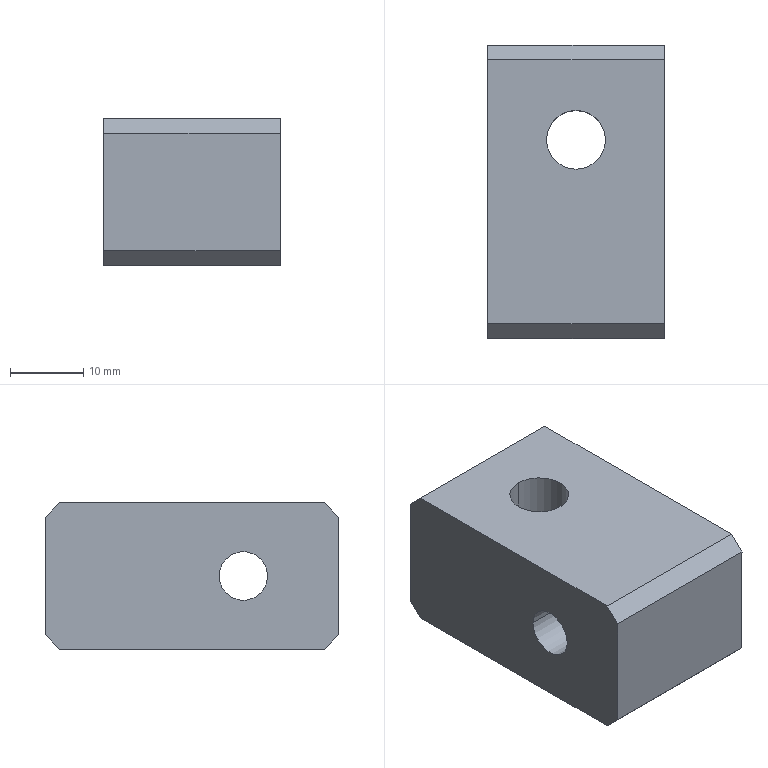Component | SolidWorks | 2SZT-2-007-2 | 1 solid | 17 faces | box 24 x 40 x 20 mm | volume 16792 mm3 | plane 11 | cylinder 6 | commonest cylinder face diameters 11 x2 6.6 x2 8 x2
build123d program:
from build123d import *

# Parameters (mm, degrees)
SKETCH1_W                                       = 40
SKETCH1_H                                       = 20
BOSS_EXTRUDE1_DEPTH                             = 24
M8X1_0_TAPPED_HOLE1_D                           = 8
M6_HEX_SOCKET_HEAD_CAP_SCREW_CBORE1_D           = 6.6
M6_HEX_SOCKET_HEAD_CAP_SCREW_CBORE1_CBORE_D     = 11
M6_HEX_SOCKET_HEAD_CAP_SCREW_CBORE1_CBORE_DEPTH = 6.4
CHAMFER1_SIZE                                   = 2


with BuildPart() as part:
    # Sketch1 → Boss-Extrude1 (new body)
    with BuildSketch(Plane(origin=(0, 0, 0), x_dir=(0, 0, -1), z_dir=(1, 0, 0))):
        with Locations((20, 10)):
            Rectangle(SKETCH1_W, SKETCH1_H)
    extrude(amount=BOSS_EXTRUDE1_DEPTH)

    # M8x1.0 Tapped Hole1 (through all)
    with Locations(Plane(origin=(0, 0, 0), x_dir=(-1, 0, 0), z_dir=(0, -1, 0))):
        with Locations((-12, 12.9)):
            Hole(M8X1_0_TAPPED_HOLE1_D / 2)

    # M6 Hex Socket Head Cap Screw CBORE1 (through all)
    with Locations(Plane(origin=(24, 0, 0), x_dir=(0, 0, -1), z_dir=(1, 0, 0))):
        with Locations((27, 10)):
            CounterBoreHole(M6_HEX_SOCKET_HEAD_CAP_SCREW_CBORE1_D / 2, M6_HEX_SOCKET_HEAD_CAP_SCREW_CBORE1_CBORE_D / 2, M6_HEX_SOCKET_HEAD_CAP_SCREW_CBORE1_CBORE_DEPTH)

    # Chamfer1
    chamfer1_edges = [part.edges().sort_by_distance(p)[0] for p in [
        (12, 20, 0),
        (12, 20, -40),
        (12, 0, -40),
        (12, 0, 0),
    ]]
    chamfer(chamfer1_edges, length=CHAMFER1_SIZE)


solid = part.part

# Placed as in the assembly
solid = solid.moved(Location((988.263, 388.093, -373.197), (-90, 0, 0)))
STEP:
#1=CARTESIAN_POINT('',(39.601,14.433,-15.087));
#2=VERTEX_POINT('',#1);
#3=CARTESIAN_POINT('',(39.601,14.,-15.087));
#4=VERTEX_POINT('',#3);
#5=CARTESIAN_POINT('',(39.601,14.216,-15.087));
#6=DIRECTION('',(1.,-0.,-0.00002551));
#7=DIRECTION('',(0.,-1.,0.));
#8=AXIS2_PLACEMENT_3D('',#5,#6,#7);
#9=CIRCLE('',#8,0.2165);
#10=EDGE_CURVE('',#2,#4,#9,.T.);
#11=ORIENTED_EDGE('',*,*,#10,.F.);
#12=CARTESIAN_POINT('',(39.853,14.433,-15.087));
#13=VERTEX_POINT('',#12);
#14=CARTESIAN_POINT('',(39.853,14.433,-15.087));
#15=DIRECTION('',(1.,-0.,-0.00002551));
#16=VECTOR('',#15,39.37);
#17=LINE('',#14,#16);
#18=EDGE_CURVE('',#2,#13,#17,.T.);
#19=ORIENTED_EDGE('',*,*,#18,.T.);
#20=CARTESIAN_POINT('',(39.853,14.,-15.087));
#21=VERTEX_POINT('',#20);
#22=CARTESIAN_POINT('',(39.853,14.216,-15.087));
#23=DIRECTION('',(1.,-0.,-0.00002551));
#24=DIRECTION('',(0.,-1.,0.));
#25=AXIS2_PLACEMENT_3D('',#22,#23,#24);
#26=CIRCLE('',#25,0.2165);
#27=EDGE_CURVE('',#13,#21,#26,.T.);
#28=ORIENTED_EDGE('',*,*,#27,.T.);
#29=CARTESIAN_POINT('',(39.853,14.,-15.087));
#30=DIRECTION('',(1.,-0.,-0.00002551));
#31=VECTOR('',#30,39.37);
#32=LINE('',#29,#31);
#33=EDGE_CURVE('',#4,#21,#32,.T.);
#34=ORIENTED_EDGE('',*,*,#33,.F.);
#35=EDGE_LOOP('',(#11,#19,#28,#34));
#36=FACE_OUTER_BOUND('',#35,.T.);
#37=CARTESIAN_POINT('',(39.853,14.216,-15.087));
#38=DIRECTION('',(1.,-0.,-0.00002551));
#39=DIRECTION('',(0.,-1.,0.));
#40=AXIS2_PLACEMENT_3D('',#37,#38,#39);
#41=CYLINDRICAL_SURFACE('',#40,0.2165);
#42=ADVANCED_FACE('',(#36),#41,.F.);
#43=CARTESIAN_POINT('',(38.908,14.346,-15.086));
#44=VERTEX_POINT('',#43);
#45=CARTESIAN_POINT('',(38.908,14.086,-15.086));
#46=VERTEX_POINT('',#45);
#47=CARTESIAN_POINT('',(38.908,14.216,-15.086));
#48=DIRECTION('',(1.,-0.,-0.00002551));
#49=DIRECTION('',(0.,-1.,0.));
#50=AXIS2_PLACEMENT_3D('',#47,#48,#49);
#51=CIRCLE('',#50,0.1299);
#52=EDGE_CURVE('',#44,#46,#51,.T.);
#53=ORIENTED_EDGE('',*,*,#52,.F.);
#54=CARTESIAN_POINT('',(39.601,14.346,-15.087));
#55=VERTEX_POINT('',#54);
#56=CARTESIAN_POINT('',(39.853,14.346,-15.087));
#57=DIRECTION('',(1.,-0.,-0.00002551));
#58=VECTOR('',#57,39.37);
#59=LINE('',#56,#58);
#60=EDGE_CURVE('',#44,#55,#59,.T.);
#61=ORIENTED_EDGE('',*,*,#60,.T.);
#62=CARTESIAN_POINT('',(39.601,14.086,-15.087));
#63=VERTEX_POINT('',#62);
#64=CARTESIAN_POINT('',(39.601,14.216,-15.087));
#65=DIRECTION('',(1.,-0.,-0.00002551));
#66=DIRECTION('',(0.,-1.,0.));
#67=AXIS2_PLACEMENT_3D('',#64,#65,#66);
#68=CIRCLE('',#67,0.1299);
#69=EDGE_CURVE('',#55,#63,#68,.T.);
#70=ORIENTED_EDGE('',*,*,#69,.T.);
#71=CARTESIAN_POINT('',(39.853,14.086,-15.087));
#72=DIRECTION('',(1.,-0.,-0.00002551));
#73=VECTOR('',#72,39.37);
#74=LINE('',#71,#73);
#75=EDGE_CURVE('',#46,#63,#74,.T.);
#76=ORIENTED_EDGE('',*,*,#75,.F.);
#77=EDGE_LOOP('',(#53,#61,#70,#76));
#78=FACE_OUTER_BOUND('',#77,.T.);
#79=CARTESIAN_POINT('',(39.853,14.216,-15.087));
#80=DIRECTION('',(1.,-0.,-0.00002551));
#81=DIRECTION('',(0.,-1.,0.));
#82=AXIS2_PLACEMENT_3D('',#79,#80,#81);
#83=CYLINDRICAL_SURFACE('',#82,0.1299);
#84=ADVANCED_FACE('',(#78),#83,.F.);
#85=CARTESIAN_POINT('',(39.38,14.929,-15.48));
#86=VERTEX_POINT('',#85);
#87=CARTESIAN_POINT('',(39.38,14.614,-15.48));
#88=VERTEX_POINT('',#87);
#89=CARTESIAN_POINT('',(39.38,14.771,-15.48));
#90=DIRECTION('',(0.00002551,0.,1.));
#91=DIRECTION('',(0.,-1.,0.));
#92=AXIS2_PLACEMENT_3D('',#89,#90,#91);
#93=CIRCLE('',#92,0.1575);
#94=EDGE_CURVE('',#86,#88,#93,.T.);
#95=ORIENTED_EDGE('',*,*,#94,.F.);
#96=CARTESIAN_POINT('',(39.38,14.929,-14.693));
#97=VERTEX_POINT('',#96);
#98=CARTESIAN_POINT('',(39.38,14.929,-14.693));
#99=DIRECTION('',(0.00002551,0.,1.));
#100=VECTOR('',#99,39.37);
#101=LINE('',#98,#100);
#102=EDGE_CURVE('',#86,#97,#101,.T.);
#103=ORIENTED_EDGE('',*,*,#102,.T.);
#104=CARTESIAN_POINT('',(39.38,14.614,-14.693));
#105=VERTEX_POINT('',#104);
#106=CARTESIAN_POINT('',(39.38,14.771,-14.693));
#107=DIRECTION('',(0.00002551,0.,1.));
#108=DIRECTION('',(0.,-1.,0.));
#109=AXIS2_PLACEMENT_3D('',#106,#107,#108);
#110=CIRCLE('',#109,0.1575);
#111=EDGE_CURVE('',#97,#105,#110,.T.);
#112=ORIENTED_EDGE('',*,*,#111,.T.);
#113=CARTESIAN_POINT('',(39.38,14.614,-14.693));
#114=DIRECTION('',(0.00002551,0.,1.));
#115=VECTOR('',#114,39.37);
#116=LINE('',#113,#115);
#117=EDGE_CURVE('',#88,#105,#116,.T.);
#118=ORIENTED_EDGE('',*,*,#117,.F.);
#119=EDGE_LOOP('',(#95,#103,#112,#118));
#120=FACE_OUTER_BOUND('',#119,.T.);
#121=CARTESIAN_POINT('',(39.38,14.771,-14.693));
#122=DIRECTION('',(0.00002551,0.,1.));
#123=DIRECTION('',(0.,-1.,0.));
#124=AXIS2_PLACEMENT_3D('',#121,#122,#123);
#125=CYLINDRICAL_SURFACE('',#124,0.1575);
#126=ADVANCED_FACE('',(#120),#125,.F.);
#127=CARTESIAN_POINT('',(39.853,15.279,-15.401));
#128=VERTEX_POINT('',#127);
#129=CARTESIAN_POINT('',(39.853,15.279,-14.772));
#130=VERTEX_POINT('',#129);
#131=CARTESIAN_POINT('',(39.853,15.279,-14.693));
#132=DIRECTION('',(0.00002551,0.,1.));
#133=VECTOR('',#132,39.37);
#134=LINE('',#131,#133);
#135=EDGE_CURVE('',#128,#130,#134,.T.);
#136=ORIENTED_EDGE('',*,*,#135,.F.);
#137=CARTESIAN_POINT('',(38.908,15.279,-15.401));
#138=VERTEX_POINT('',#137);
#139=CARTESIAN_POINT('',(39.853,15.279,-15.401));
#140=DIRECTION('',(-1.,0.,0.00002551));
#141=VECTOR('',#140,39.37);
#142=LINE('',#139,#141);
#143=EDGE_CURVE('',#128,#138,#142,.T.);
#144=ORIENTED_EDGE('',*,*,#143,.T.);
#145=CARTESIAN_POINT('',(38.908,15.279,-14.772));
#146=VERTEX_POINT('',#145);
#147=CARTESIAN_POINT('',(38.908,15.279,-14.693));
#148=DIRECTION('',(0.00002551,0.,1.));
#149=VECTOR('',#148,39.37);
#150=LINE('',#147,#149);
#151=EDGE_CURVE('',#138,#146,#150,.T.);
#152=ORIENTED_EDGE('',*,*,#151,.T.);
#153=CARTESIAN_POINT('',(39.853,15.279,-14.772));
#154=DIRECTION('',(1.,-0.,-0.00002551));
#155=VECTOR('',#154,39.37);
#156=LINE('',#153,#155);
#157=EDGE_CURVE('',#146,#130,#156,.T.);
#158=ORIENTED_EDGE('',*,*,#157,.T.);
#159=EDGE_LOOP('',(#136,#144,#152,#158));
#160=FACE_OUTER_BOUND('',#159,.T.);
#161=CARTESIAN_POINT('',(39.853,15.279,-14.693));
#162=DIRECTION('',(-0.,-1.,0.));
#163=DIRECTION('',(-1.,0.,0.00002551));
#164=AXIS2_PLACEMENT_3D('',#161,#162,#163);
#165=PLANE('',#164);
#166=ADVANCED_FACE('',(#160),#165,.F.);
#167=CARTESIAN_POINT('',(39.38,14.771,-14.693));
#168=DIRECTION('',(0.00002551,0.,1.));
#169=DIRECTION('',(0.,-1.,0.));
#170=AXIS2_PLACEMENT_3D('',#167,#168,#169);
#171=CIRCLE('',#170,0.1575);
#172=EDGE_CURVE('',#105,#97,#171,.T.);
#173=ORIENTED_EDGE('',*,*,#172,.F.);
#174=ORIENTED_EDGE('',*,*,#111,.F.);
#175=EDGE_LOOP('',(#173,#174));
#176=FACE_BOUND('',#175,.T.);
#177=CARTESIAN_POINT('',(38.908,15.201,-14.693));
#178=VERTEX_POINT('',#177);
#179=CARTESIAN_POINT('',(38.908,13.783,-14.693));
#180=VERTEX_POINT('',#179);
#181=CARTESIAN_POINT('',(38.908,15.279,-14.693));
#182=DIRECTION('',(-0.,-1.,0.));
#183=VECTOR('',#182,39.37);
#184=LINE('',#181,#183);
#185=EDGE_CURVE('',#178,#180,#184,.T.);
#186=ORIENTED_EDGE('',*,*,#185,.T.);
#187=CARTESIAN_POINT('',(39.853,13.783,-14.693));
#188=VERTEX_POINT('',#187);
#189=CARTESIAN_POINT('',(39.853,13.783,-14.693));
#190=DIRECTION('',(1.,-0.,-0.00002551));
#191=VECTOR('',#190,39.37);
#192=LINE('',#189,#191);
#193=EDGE_CURVE('',#180,#188,#192,.T.);
#194=ORIENTED_EDGE('',*,*,#193,.T.);
#195=CARTESIAN_POINT('',(39.853,15.201,-14.693));
#196=VERTEX_POINT('',#195);
#197=CARTESIAN_POINT('',(39.853,15.279,-14.693));
#198=DIRECTION('',(-0.,-1.,0.));
#199=VECTOR('',#198,39.37);
#200=LINE('',#197,#199);
#201=EDGE_CURVE('',#196,#188,#200,.T.);
#202=ORIENTED_EDGE('',*,*,#201,.F.);
#203=CARTESIAN_POINT('',(39.853,15.201,-14.693));
#204=DIRECTION('',(-1.,0.,0.00002551));
#205=VECTOR('',#204,39.37);
#206=LINE('',#203,#205);
#207=EDGE_CURVE('',#196,#178,#206,.T.);
#208=ORIENTED_EDGE('',*,*,#207,.T.);
#209=EDGE_LOOP('',(#186,#194,#202,#208));
#210=FACE_OUTER_BOUND('',#209,.T.);
#211=CARTESIAN_POINT('',(39.853,15.279,-14.693));
#212=DIRECTION('',(-0.00002551,-0.,-1.));
#213=DIRECTION('',(0.,1.,-0.));
#214=AXIS2_PLACEMENT_3D('',#211,#212,#213);
#215=PLANE('',#214);
#216=ADVANCED_FACE('',(#176,#210),#215,.F.);
#217=CARTESIAN_POINT('',(38.908,13.704,-14.772));
#218=VERTEX_POINT('',#217);
#219=CARTESIAN_POINT('',(38.908,13.704,-15.401));
#220=VERTEX_POINT('',#219);
#221=CARTESIAN_POINT('',(38.908,13.704,-14.693));
#222=DIRECTION('',(-0.00002551,-0.,-1.));
#223=VECTOR('',#222,39.37);
#224=LINE('',#221,#223);
#225=EDGE_CURVE('',#218,#220,#224,.T.);
#226=ORIENTED_EDGE('',*,*,#225,.T.);
#227=CARTESIAN_POINT('',(39.853,13.704,-15.401));
#228=VERTEX_POINT('',#227);
#229=CARTESIAN_POINT('',(39.853,13.704,-15.401));
#230=DIRECTION('',(1.,-0.,-0.00002551));
#231=VECTOR('',#230,39.37);
#232=LINE('',#229,#231);
#233=EDGE_CURVE('',#220,#228,#232,.T.);
#234=ORIENTED_EDGE('',*,*,#233,.T.);
#235=CARTESIAN_POINT('',(39.853,13.704,-14.772));
#236=VERTEX_POINT('',#235);
#237=CARTESIAN_POINT('',(39.853,13.704,-14.693));
#238=DIRECTION('',(-0.00002551,-0.,-1.));
#239=VECTOR('',#238,39.37);
#240=LINE('',#237,#239);
#241=EDGE_CURVE('',#236,#228,#240,.T.);
#242=ORIENTED_EDGE('',*,*,#241,.F.);
#243=CARTESIAN_POINT('',(39.853,13.704,-14.772));
#244=DIRECTION('',(-1.,0.,0.00002551));
#245=VECTOR('',#244,39.37);
#246=LINE('',#243,#245);
#247=EDGE_CURVE('',#236,#218,#246,.T.);
#248=ORIENTED_EDGE('',*,*,#247,.T.);
#249=EDGE_LOOP('',(#226,#234,#242,#248));
#250=FACE_OUTER_BOUND('',#249,.T.);
#251=CARTESIAN_POINT('',(39.853,13.704,-14.693));
#252=DIRECTION('',(0.,1.,-0.));
#253=DIRECTION('',(1.,-0.,-0.00002551));
#254=AXIS2_PLACEMENT_3D('',#251,#252,#253);
#255=PLANE('',#254);
#256=ADVANCED_FACE('',(#250),#255,.F.);
#257=CARTESIAN_POINT('',(39.38,14.771,-15.48));
#258=DIRECTION('',(0.00002551,0.,1.));
#259=DIRECTION('',(0.,-1.,0.));
#260=AXIS2_PLACEMENT_3D('',#257,#258,#259);
#261=CIRCLE('',#260,0.1575);
#262=EDGE_CURVE('',#88,#86,#261,.T.);
#263=ORIENTED_EDGE('',*,*,#262,.T.);
#264=ORIENTED_EDGE('',*,*,#94,.T.);
#265=EDGE_LOOP('',(#263,#264));
#266=FACE_BOUND('',#265,.T.);
#267=CARTESIAN_POINT('',(39.853,13.783,-15.48));
#268=VERTEX_POINT('',#267);
#269=CARTESIAN_POINT('',(39.853,15.201,-15.48));
#270=VERTEX_POINT('',#269);
#271=CARTESIAN_POINT('',(39.853,15.279,-15.48));
#272=DIRECTION('',(0.,1.,-0.));
#273=VECTOR('',#272,39.37);
#274=LINE('',#271,#273);
#275=EDGE_CURVE('',#268,#270,#274,.T.);
#276=ORIENTED_EDGE('',*,*,#275,.F.);
#277=CARTESIAN_POINT('',(38.908,13.783,-15.48));
#278=VERTEX_POINT('',#277);
#279=CARTESIAN_POINT('',(39.853,13.783,-15.48));
#280=DIRECTION('',(-1.,0.,0.00002551));
#281=VECTOR('',#280,39.37);
#282=LINE('',#279,#281);
#283=EDGE_CURVE('',#268,#278,#282,.T.);
#284=ORIENTED_EDGE('',*,*,#283,.T.);
#285=CARTESIAN_POINT('',(38.908,15.201,-15.48));
#286=VERTEX_POINT('',#285);
#287=CARTESIAN_POINT('',(38.908,15.279,-15.48));
#288=DIRECTION('',(0.,1.,-0.));
#289=VECTOR('',#288,39.37);
#290=LINE('',#287,#289);
#291=EDGE_CURVE('',#278,#286,#290,.T.);
#292=ORIENTED_EDGE('',*,*,#291,.T.);
#293=CARTESIAN_POINT('',(39.853,15.201,-15.48));
#294=DIRECTION('',(1.,-0.,-0.00002551));
#295=VECTOR('',#294,39.37);
#296=LINE('',#293,#295);
#297=EDGE_CURVE('',#286,#270,#296,.T.);
#298=ORIENTED_EDGE('',*,*,#297,.T.);
#299=EDGE_LOOP('',(#276,#284,#292,#298));
#300=FACE_OUTER_BOUND('',#299,.T.);
#301=CARTESIAN_POINT('',(39.853,15.279,-15.48));
#302=DIRECTION('',(0.00002551,0.,1.));
#303=DIRECTION('',(-0.,-1.,0.));
#304=AXIS2_PLACEMENT_3D('',#301,#302,#303);
#305=PLANE('',#304);
#306=ADVANCED_FACE('',(#266,#300),#305,.F.);
#307=CARTESIAN_POINT('',(39.853,14.216,-15.087));
#308=DIRECTION('',(1.,-0.,-0.00002551));
#309=DIRECTION('',(0.,-1.,0.));
#310=AXIS2_PLACEMENT_3D('',#307,#308,#309);
#311=CIRCLE('',#310,0.2165);
#312=EDGE_CURVE('',#21,#13,#311,.T.);
#313=ORIENTED_EDGE('',*,*,#312,.F.);
#314=ORIENTED_EDGE('',*,*,#27,.F.);
#315=EDGE_LOOP('',(#313,#314));
#316=FACE_BOUND('',#315,.T.);
#317=ORIENTED_EDGE('',*,*,#241,.T.);
#318=CARTESIAN_POINT('',(39.853,13.783,-15.48));
#319=DIRECTION('',(-0.00001804,0.7071,-0.7071));
#320=VECTOR('',#319,39.37);
#321=LINE('',#318,#320);
#322=EDGE_CURVE('',#228,#268,#321,.T.);
#323=ORIENTED_EDGE('',*,*,#322,.T.);
#324=ORIENTED_EDGE('',*,*,#275,.T.);
#325=CARTESIAN_POINT('',(39.853,15.279,-15.401));
#326=DIRECTION('',(0.00001804,0.7071,0.7071));
#327=VECTOR('',#326,39.37);
#328=LINE('',#325,#327);
#329=EDGE_CURVE('',#270,#128,#328,.T.);
#330=ORIENTED_EDGE('',*,*,#329,.T.);
#331=ORIENTED_EDGE('',*,*,#135,.T.);
#332=CARTESIAN_POINT('',(39.853,15.201,-14.693));
#333=DIRECTION('',(0.00001804,-0.7071,0.7071));
#334=VECTOR('',#333,39.37);
#335=LINE('',#332,#334);
#336=EDGE_CURVE('',#130,#196,#335,.T.);
#337=ORIENTED_EDGE('',*,*,#336,.T.);
#338=ORIENTED_EDGE('',*,*,#201,.T.);
#339=CARTESIAN_POINT('',(39.853,13.704,-14.772));
#340=DIRECTION('',(-0.00001804,-0.7071,-0.7071));
#341=VECTOR('',#340,39.37);
#342=LINE('',#339,#341);
#343=EDGE_CURVE('',#188,#236,#342,.T.);
#344=ORIENTED_EDGE('',*,*,#343,.T.);
#345=EDGE_LOOP('',(#317,#323,#324,#330,#331,#337,#338,#344));
#346=FACE_OUTER_BOUND('',#345,.T.);
#347=CARTESIAN_POINT('',(39.853,15.279,-14.693));
#348=DIRECTION('',(-1.,0.,0.00002551));
#349=DIRECTION('',(0.,1.,-0.));
#350=AXIS2_PLACEMENT_3D('',#347,#348,#349);
#351=PLANE('',#350);
#352=ADVANCED_FACE('',(#316,#346),#351,.F.);
#353=CARTESIAN_POINT('',(38.908,14.216,-15.086));
#354=DIRECTION('',(1.,-0.,-0.00002551));
#355=DIRECTION('',(0.,-1.,0.));
#356=AXIS2_PLACEMENT_3D('',#353,#354,#355);
#357=CIRCLE('',#356,0.1299);
#358=EDGE_CURVE('',#46,#44,#357,.T.);
#359=ORIENTED_EDGE('',*,*,#358,.T.);
#360=ORIENTED_EDGE('',*,*,#52,.T.);
#361=EDGE_LOOP('',(#359,#360));
#362=FACE_BOUND('',#361,.T.);
#363=ORIENTED_EDGE('',*,*,#291,.F.);
#364=CARTESIAN_POINT('',(38.908,14.138,-15.835));
#365=DIRECTION('',(0.00001804,-0.7071,0.7071));
#366=VECTOR('',#365,39.37);
#367=LINE('',#364,#366);
#368=EDGE_CURVE('',#278,#220,#367,.T.);
#369=ORIENTED_EDGE('',*,*,#368,.T.);
#370=ORIENTED_EDGE('',*,*,#225,.F.);
#371=CARTESIAN_POINT('',(38.908,14.531,-13.945));
#372=DIRECTION('',(0.00001804,0.7071,0.7071));
#373=VECTOR('',#372,39.37);
#374=LINE('',#371,#373);
#375=EDGE_CURVE('',#218,#180,#374,.T.);
#376=ORIENTED_EDGE('',*,*,#375,.T.);
#377=ORIENTED_EDGE('',*,*,#185,.F.);
#378=CARTESIAN_POINT('',(38.908,15.24,-14.732));
#379=DIRECTION('',(-0.00001804,0.7071,-0.7071));
#380=VECTOR('',#379,39.37);
#381=LINE('',#378,#380);
#382=EDGE_CURVE('',#178,#146,#381,.T.);
#383=ORIENTED_EDGE('',*,*,#382,.T.);
#384=ORIENTED_EDGE('',*,*,#151,.F.);
#385=CARTESIAN_POINT('',(38.908,15.634,-15.047));
#386=DIRECTION('',(-0.00001804,-0.7071,-0.7071));
#387=VECTOR('',#386,39.37);
#388=LINE('',#385,#387);
#389=EDGE_CURVE('',#138,#286,#388,.T.);
#390=ORIENTED_EDGE('',*,*,#389,.T.);
#391=EDGE_LOOP('',(#363,#369,#370,#376,#377,#383,#384,#390));
#392=FACE_OUTER_BOUND('',#391,.T.);
#393=CARTESIAN_POINT('',(38.908,15.279,-14.693));
#394=DIRECTION('',(-1.,0.,0.00002551));
#395=DIRECTION('',(0.,1.,-0.));
#396=AXIS2_PLACEMENT_3D('',#393,#394,#395);
#397=PLANE('',#396);
#398=ADVANCED_FACE('',(#362,#392),#397,.T.);
#399=ORIENTED_EDGE('',*,*,#102,.F.);
#400=ORIENTED_EDGE('',*,*,#262,.F.);
#401=ORIENTED_EDGE('',*,*,#117,.T.);
#402=ORIENTED_EDGE('',*,*,#172,.T.);
#403=EDGE_LOOP('',(#399,#400,#401,#402));
#404=FACE_OUTER_BOUND('',#403,.T.);
#405=CARTESIAN_POINT('',(39.38,14.771,-14.693));
#406=DIRECTION('',(0.00002551,0.,1.));
#407=DIRECTION('',(0.,-1.,0.));
#408=AXIS2_PLACEMENT_3D('',#405,#406,#407);
#409=CYLINDRICAL_SURFACE('',#408,0.1575);
#410=ADVANCED_FACE('',(#404),#409,.F.);
#411=ORIENTED_EDGE('',*,*,#60,.F.);
#412=ORIENTED_EDGE('',*,*,#358,.F.);
#413=ORIENTED_EDGE('',*,*,#75,.T.);
#414=CARTESIAN_POINT('',(39.601,14.216,-15.087));
#415=DIRECTION('',(1.,-0.,-0.00002551));
#416=DIRECTION('',(0.,-1.,0.));
#417=AXIS2_PLACEMENT_3D('',#414,#415,#416);
#418=CIRCLE('',#417,0.1299);
#419=EDGE_CURVE('',#63,#55,#418,.T.);
#420=ORIENTED_EDGE('',*,*,#419,.T.);
#421=EDGE_LOOP('',(#411,#412,#413,#420));
#422=FACE_OUTER_BOUND('',#421,.T.);
#423=CARTESIAN_POINT('',(39.853,14.216,-15.087));
#424=DIRECTION('',(1.,-0.,-0.00002551));
#425=DIRECTION('',(0.,-1.,0.));
#426=AXIS2_PLACEMENT_3D('',#423,#424,#425);
#427=CYLINDRICAL_SURFACE('',#426,0.1299);
#428=ADVANCED_FACE('',(#422),#427,.F.);
#429=ORIENTED_EDGE('',*,*,#419,.F.);
#430=ORIENTED_EDGE('',*,*,#69,.F.);
#431=EDGE_LOOP('',(#429,#430));
#432=FACE_BOUND('',#431,.T.);
#433=CARTESIAN_POINT('',(39.601,14.216,-15.087));
#434=DIRECTION('',(1.,-0.,-0.00002551));
#435=DIRECTION('',(0.,-1.,0.));
#436=AXIS2_PLACEMENT_3D('',#433,#434,#435);
#437=CIRCLE('',#436,0.2165);
#438=EDGE_CURVE('',#4,#2,#437,.T.);
#439=ORIENTED_EDGE('',*,*,#438,.T.);
#440=ORIENTED_EDGE('',*,*,#10,.T.);
#441=EDGE_LOOP('',(#439,#440));
#442=FACE_OUTER_BOUND('',#441,.T.);
#443=CARTESIAN_POINT('',(39.601,14.216,-15.216));
#444=DIRECTION('',(-1.,0.,0.00002551));
#445=DIRECTION('',(0.,1.,-0.));
#446=AXIS2_PLACEMENT_3D('',#443,#444,#445);
#447=PLANE('',#446);
#448=ADVANCED_FACE('',(#432,#442),#447,.F.);
#449=ORIENTED_EDGE('',*,*,#18,.F.);
#450=ORIENTED_EDGE('',*,*,#438,.F.);
#451=ORIENTED_EDGE('',*,*,#33,.T.);
#452=ORIENTED_EDGE('',*,*,#312,.T.);
#453=EDGE_LOOP('',(#449,#450,#451,#452));
#454=FACE_OUTER_BOUND('',#453,.T.);
#455=CARTESIAN_POINT('',(39.853,14.216,-15.087));
#456=DIRECTION('',(1.,-0.,-0.00002551));
#457=DIRECTION('',(0.,-1.,0.));
#458=AXIS2_PLACEMENT_3D('',#455,#456,#457);
#459=CYLINDRICAL_SURFACE('',#458,0.2165);
#460=ADVANCED_FACE('',(#454),#459,.F.);
#461=ORIENTED_EDGE('',*,*,#322,.F.);
#462=ORIENTED_EDGE('',*,*,#233,.F.);
#463=ORIENTED_EDGE('',*,*,#368,.F.);
#464=ORIENTED_EDGE('',*,*,#283,.F.);
#465=EDGE_LOOP('',(#461,#462,#463,#464));
#466=FACE_OUTER_BOUND('',#465,.T.);
#467=CARTESIAN_POINT('',(39.853,13.783,-15.48));
#468=DIRECTION('',(0.00001804,0.7071,0.7071));
#469=DIRECTION('',(-1.,0.,0.00002551));
#470=AXIS2_PLACEMENT_3D('',#467,#468,#469);
#471=PLANE('',#470);
#472=ADVANCED_FACE('',(#466),#471,.F.);
#473=ORIENTED_EDGE('',*,*,#343,.F.);
#474=ORIENTED_EDGE('',*,*,#193,.F.);
#475=ORIENTED_EDGE('',*,*,#375,.F.);
#476=ORIENTED_EDGE('',*,*,#247,.F.);
#477=EDGE_LOOP('',(#473,#474,#475,#476));
#478=FACE_OUTER_BOUND('',#477,.T.);
#479=CARTESIAN_POINT('',(39.853,13.704,-14.772));
#480=DIRECTION('',(-0.00001804,0.7071,-0.7071));
#481=DIRECTION('',(-1.,0.,0.00002551));
#482=AXIS2_PLACEMENT_3D('',#479,#480,#481);
#483=PLANE('',#482);
#484=ADVANCED_FACE('',(#478),#483,.F.);
#485=ORIENTED_EDGE('',*,*,#329,.F.);
#486=ORIENTED_EDGE('',*,*,#297,.F.);
#487=ORIENTED_EDGE('',*,*,#389,.F.);
#488=ORIENTED_EDGE('',*,*,#143,.F.);
#489=EDGE_LOOP('',(#485,#486,#487,#488));
#490=FACE_OUTER_BOUND('',#489,.T.);
#491=CARTESIAN_POINT('',(39.853,15.279,-15.401));
#492=DIRECTION('',(0.00001804,-0.7071,0.7071));
#493=DIRECTION('',(-1.,0.,0.00002551));
#494=AXIS2_PLACEMENT_3D('',#491,#492,#493);
#495=PLANE('',#494);
#496=ADVANCED_FACE('',(#490),#495,.F.);
#497=ORIENTED_EDGE('',*,*,#336,.F.);
#498=ORIENTED_EDGE('',*,*,#157,.F.);
#499=ORIENTED_EDGE('',*,*,#382,.F.);
#500=ORIENTED_EDGE('',*,*,#207,.F.);
#501=EDGE_LOOP('',(#497,#498,#499,#500));
#502=FACE_OUTER_BOUND('',#501,.T.);
#503=CARTESIAN_POINT('',(39.853,15.201,-14.693));
#504=DIRECTION('',(-0.00001804,-0.7071,-0.7071));
#505=DIRECTION('',(-1.,0.,0.00002551));
#506=AXIS2_PLACEMENT_3D('',#503,#504,#505);
#507=PLANE('',#506);
#508=ADVANCED_FACE('',(#502),#507,.F.);
#509=CLOSED_SHELL('',(#42,#84,#126,#166,#216,#256,#306,#352,#398,#410,#428,#448,#460,#472,#484,#496,#508));
#510=MANIFOLD_SOLID_BREP('',#509);
#511=CARTESIAN_POINT('',(0.,0.,0.));
#512=DIRECTION('',(0.,0.,1.));
#513=DIRECTION('',(1.,0.,0.));
#514=AXIS2_PLACEMENT_3D('',#511,#512,#513);
#515=(LENGTH_UNIT()NAMED_UNIT(*)SI_UNIT($,.METRE.));
#516=LENGTH_MEASURE_WITH_UNIT(LENGTH_MEASURE(0.0254),#515);
#517=DIMENSIONAL_EXPONENTS(1.,0.,0.,0.,0.,0.,0.);
#518=(CONVERSION_BASED_UNIT('',#516)LENGTH_UNIT()NAMED_UNIT(#517));
#519=UNCERTAINTY_MEASURE_WITH_UNIT(LENGTH_MEASURE(0.00001),#518,'','');
#520=(NAMED_UNIT(*)PLANE_ANGLE_UNIT()SI_UNIT($,.RADIAN.));
#521=(NAMED_UNIT(*)SI_UNIT($,.STERADIAN.)SOLID_ANGLE_UNIT());
#522=(GEOMETRIC_REPRESENTATION_CONTEXT(3)GLOBAL_UNCERTAINTY_ASSIGNED_CONTEXT((#519))GLOBAL_UNIT_ASSIGNED_CONTEXT((#518,#520,#521))REPRESENTATION_CONTEXT('',''));
#523=ADVANCED_BREP_SHAPE_REPRESENTATION('',(#510,#514),#522);
#524=COLOUR_RGB('',0.7922,0.8196,0.9333);
#525=FILL_AREA_STYLE_COLOUR('',#524);
#526=FILL_AREA_STYLE('',(#525));
#527=SURFACE_STYLE_FILL_AREA(#526);
#528=SURFACE_SIDE_STYLE('',(#527));
#529=SURFACE_STYLE_USAGE(.BOTH.,#528);
#530=PRESENTATION_STYLE_ASSIGNMENT((#529));
#531=STYLED_ITEM('',(#530),#510);
#532=PRESENTATION_LAYER_ASSIGNMENT('','',(#531));
#533=(LENGTH_UNIT()NAMED_UNIT(*)SI_UNIT($,.METRE.));
#534=LENGTH_MEASURE_WITH_UNIT(LENGTH_MEASURE(0.0254),#533);
#535=DIMENSIONAL_EXPONENTS(1.,0.,0.,0.,0.,0.,0.);
#536=(CONVERSION_BASED_UNIT('',#534)LENGTH_UNIT()NAMED_UNIT(#535));
#537=UNCERTAINTY_MEASURE_WITH_UNIT(LENGTH_MEASURE(0.00001),#536,'','');
#538=(NAMED_UNIT(*)PLANE_ANGLE_UNIT()SI_UNIT($,.RADIAN.));
#539=(NAMED_UNIT(*)SI_UNIT($,.STERADIAN.)SOLID_ANGLE_UNIT());
#540=(GEOMETRIC_REPRESENTATION_CONTEXT(3)GLOBAL_UNCERTAINTY_ASSIGNED_CONTEXT((#537))GLOBAL_UNIT_ASSIGNED_CONTEXT((#536,#538,#539))REPRESENTATION_CONTEXT('',''));
#541=MECHANICAL_DESIGN_GEOMETRIC_PRESENTATION_REPRESENTATION('',(#531),#540);